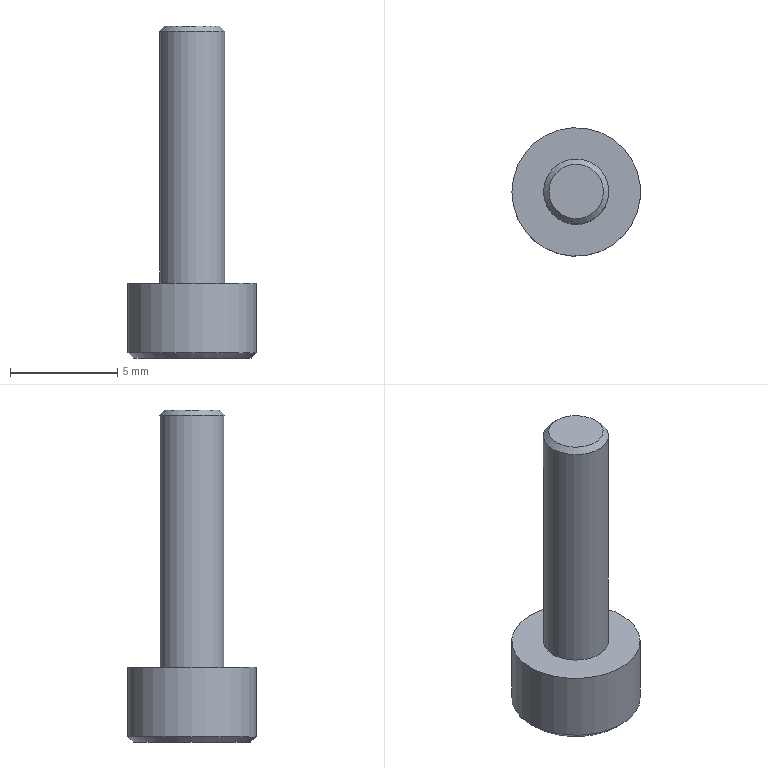Component | NX | SCREW_1 | 1 solid | 14 faces | box 6 x 6 x 15.5 mm | volume 158 mm3 | plane 10 | cylinder 2 | cone 2 | commonest cylinder face diameters 3.045 x1 6 x1
STEP:
#1=CARTESIAN_POINT('',(0.,0.,0.));
#2=DIRECTION('',(0.,0.,1.));
#3=DIRECTION('',(1.,0.,0.));
#4=AXIS2_PLACEMENT_3D('',#1,#2,#3);
#5=CARTESIAN_POINT('',(21.273,19.,-19.));
#6=VERTEX_POINT('',#5);
#7=CARTESIAN_POINT('',(20.,19.,-19.));
#8=DIRECTION('',(0.,0.,1.));
#9=DIRECTION('',(1.,0.,0.));
#10=AXIS2_PLACEMENT_3D('',#7,#8,#9);
#11=CIRCLE('',#10,1.273);
#12=CARTESIAN_POINT('',(20.,19.,-19.));
#13=DIRECTION('',(0.,0.,1.));
#14=DIRECTION('',(1.,0.,0.));
#15=AXIS2_PLACEMENT_3D('',#12,#13,#14);
#16=PLANE('',#15);
#17=CARTESIAN_POINT('',(0.,0.));
#18=DIRECTION('',(1.,0.));
#19=AXIS2_PLACEMENT_2D('',#17,#18);
#20=CIRCLE('',#19,1.273);
#21=(GEOMETRIC_REPRESENTATION_CONTEXT(2)PARAMETRIC_REPRESENTATION_CONTEXT()REPRESENTATION_CONTEXT('',''));
#22=DEFINITIONAL_REPRESENTATION('',(#20),#21);
#23=PCURVE('',#16,#22);
#24=CARTESIAN_POINT('',(20.,19.,-19.25));
#25=DIRECTION('',(0.,0.,-1.));
#26=DIRECTION('',(-1.,0.,0.));
#27=AXIS2_PLACEMENT_3D('',#24,#25,#26);
#28=CONICAL_SURFACE('',#27,1.523,0.7854);
#29=CARTESIAN_POINT('',(9.425,-0.25));
#30=DIRECTION('',(-1.,0.));
#31=VECTOR('',#30,1.);
#32=LINE('',#29,#31);
#33=(GEOMETRIC_REPRESENTATION_CONTEXT(2)PARAMETRIC_REPRESENTATION_CONTEXT()REPRESENTATION_CONTEXT('',''));
#34=DEFINITIONAL_REPRESENTATION('',(#32),#33);
#35=PCURVE('',#28,#34);
#36=SURFACE_CURVE('',#11,(#23,#35),.PCURVE_S1.);
#37=EDGE_CURVE('',#6,#6,#36,.T.);
#38=ORIENTED_EDGE('',*,*,#37,.T.);
#39=EDGE_LOOP('',(#38));
#40=FACE_BOUND('',#39,.T.);
#41=ADVANCED_FACE('',(#40),#16,.T.);
#42=CARTESIAN_POINT('',(21.523,19.,-19.25));
#43=VERTEX_POINT('',#42);
#44=CARTESIAN_POINT('',(18.477,19.,-19.25));
#45=VERTEX_POINT('',#44);
#46=CARTESIAN_POINT('',(20.,19.,-19.25));
#47=DIRECTION('',(0.,0.,-1.));
#48=DIRECTION('',(1.,0.,0.));
#49=AXIS2_PLACEMENT_3D('',#46,#47,#48);
#50=CIRCLE('',#49,1.523);
#51=CARTESIAN_POINT('',(20.,19.,-19.));
#52=DIRECTION('',(0.,0.,-1.));
#53=DIRECTION('',(-1.,0.,0.));
#54=AXIS2_PLACEMENT_3D('',#51,#52,#53);
#55=CYLINDRICAL_SURFACE('',#54,1.523);
#56=CARTESIAN_POINT('',(3.142,0.25));
#57=DIRECTION('',(1.,0.));
#58=VECTOR('',#57,1.);
#59=LINE('',#56,#58);
#60=(GEOMETRIC_REPRESENTATION_CONTEXT(2)PARAMETRIC_REPRESENTATION_CONTEXT()REPRESENTATION_CONTEXT('',''));
#61=DEFINITIONAL_REPRESENTATION('',(#59),#60);
#62=PCURVE('',#55,#61);
#63=CARTESIAN_POINT('',(3.142,-0.));
#64=DIRECTION('',(1.,0.));
#65=VECTOR('',#64,1.);
#66=LINE('',#63,#65);
#67=(GEOMETRIC_REPRESENTATION_CONTEXT(2)PARAMETRIC_REPRESENTATION_CONTEXT()REPRESENTATION_CONTEXT('',''));
#68=DEFINITIONAL_REPRESENTATION('',(#66),#67);
#69=PCURVE('',#28,#68);
#70=SURFACE_CURVE('',#50,(#62,#69),.PCURVE_S1.);
#71=EDGE_CURVE('',#43,#45,#70,.T.);
#72=ORIENTED_EDGE('',*,*,#71,.T.);
#73=CARTESIAN_POINT('',(18.477,19.,-31.));
#74=VERTEX_POINT('',#73);
#75=CARTESIAN_POINT('',(18.477,19.,-19.25));
#76=CARTESIAN_POINT('',(18.477,19.,-31.));
#77=B_SPLINE_CURVE_WITH_KNOTS('',1,(#75,#76),.UNSPECIFIED.,.F.,.F.,(2,2),(0.25,12.),.PIECEWISE_BEZIER_KNOTS.);
#78=CARTESIAN_POINT('',(6.283,0.));
#79=DIRECTION('',(0.,1.));
#80=VECTOR('',#79,1.);
#81=LINE('',#78,#80);
#82=(GEOMETRIC_REPRESENTATION_CONTEXT(2)PARAMETRIC_REPRESENTATION_CONTEXT()REPRESENTATION_CONTEXT('',''));
#83=DEFINITIONAL_REPRESENTATION('',(#81),#82);
#84=PCURVE('',#55,#83);
#85=CARTESIAN_POINT('',(0.,0.));
#86=DIRECTION('',(0.,1.));
#87=VECTOR('',#86,1.);
#88=LINE('',#85,#87);
#89=(GEOMETRIC_REPRESENTATION_CONTEXT(2)PARAMETRIC_REPRESENTATION_CONTEXT()REPRESENTATION_CONTEXT('',''));
#90=DEFINITIONAL_REPRESENTATION('',(#88),#89);
#91=PCURVE('',#55,#90);
#92=SEAM_CURVE('',#77,(#84,#91),.PCURVE_S1.);
#93=EDGE_CURVE('',#45,#74,#92,.T.);
#94=ORIENTED_EDGE('',*,*,#93,.T.);
#95=CARTESIAN_POINT('',(20.,19.,-31.));
#96=DIRECTION('',(0.,0.,1.));
#97=DIRECTION('',(-1.,0.,0.));
#98=AXIS2_PLACEMENT_3D('',#95,#96,#97);
#99=CIRCLE('',#98,1.523);
#100=CARTESIAN_POINT('',(6.283,12.));
#101=DIRECTION('',(-1.,0.));
#102=VECTOR('',#101,1.);
#103=LINE('',#100,#102);
#104=(GEOMETRIC_REPRESENTATION_CONTEXT(2)PARAMETRIC_REPRESENTATION_CONTEXT()REPRESENTATION_CONTEXT('',''));
#105=DEFINITIONAL_REPRESENTATION('',(#103),#104);
#106=PCURVE('',#55,#105);
#107=CARTESIAN_POINT('',(20.,19.,-31.));
#108=DIRECTION('',(0.,0.,1.));
#109=DIRECTION('',(1.,0.,0.));
#110=AXIS2_PLACEMENT_3D('',#107,#108,#109);
#111=PLANE('',#110);
#112=CARTESIAN_POINT('',(0.,0.));
#113=DIRECTION('',(-1.,0.));
#114=AXIS2_PLACEMENT_2D('',#112,#113);
#115=CIRCLE('',#114,1.523);
#116=(GEOMETRIC_REPRESENTATION_CONTEXT(2)PARAMETRIC_REPRESENTATION_CONTEXT()REPRESENTATION_CONTEXT('',''));
#117=DEFINITIONAL_REPRESENTATION('',(#115),#116);
#118=PCURVE('',#111,#117);
#119=SURFACE_CURVE('',#99,(#106,#118),.PCURVE_S1.);
#120=EDGE_CURVE('',#74,#74,#119,.T.);
#121=ORIENTED_EDGE('',*,*,#120,.T.);
#122=ORIENTED_EDGE('',*,*,#93,.F.);
#123=CARTESIAN_POINT('',(20.,19.,-19.25));
#124=DIRECTION('',(0.,0.,-1.));
#125=DIRECTION('',(1.,0.,0.));
#126=AXIS2_PLACEMENT_3D('',#123,#124,#125);
#127=CIRCLE('',#126,1.523);
#128=CARTESIAN_POINT('',(-3.142,0.25));
#129=DIRECTION('',(1.,0.));
#130=VECTOR('',#129,1.);
#131=LINE('',#128,#130);
#132=(GEOMETRIC_REPRESENTATION_CONTEXT(2)PARAMETRIC_REPRESENTATION_CONTEXT()REPRESENTATION_CONTEXT('',''));
#133=DEFINITIONAL_REPRESENTATION('',(#131),#132);
#134=PCURVE('',#55,#133);
#135=CARTESIAN_POINT('',(3.142,-0.));
#136=DIRECTION('',(1.,0.));
#137=VECTOR('',#136,1.);
#138=LINE('',#135,#137);
#139=(GEOMETRIC_REPRESENTATION_CONTEXT(2)PARAMETRIC_REPRESENTATION_CONTEXT()REPRESENTATION_CONTEXT('',''));
#140=DEFINITIONAL_REPRESENTATION('',(#138),#139);
#141=PCURVE('',#28,#140);
#142=SURFACE_CURVE('',#127,(#134,#141),.PCURVE_S1.);
#143=EDGE_CURVE('',#45,#43,#142,.T.);
#144=ORIENTED_EDGE('',*,*,#143,.T.);
#145=EDGE_LOOP('',(#72,#94,#121,#122,#144));
#146=FACE_BOUND('',#145,.T.);
#147=ADVANCED_FACE('',(#146),#55,.T.);
#148=CARTESIAN_POINT('',(17.25,19.,-34.5));
#149=VERTEX_POINT('',#148);
#150=CARTESIAN_POINT('',(20.,19.,-34.5));
#151=DIRECTION('',(0.,0.,-1.));
#152=DIRECTION('',(-1.,0.,0.));
#153=AXIS2_PLACEMENT_3D('',#150,#151,#152);
#154=CIRCLE('',#153,2.75);
#155=CARTESIAN_POINT('',(20.,19.,-34.5));
#156=DIRECTION('',(0.,0.,-1.));
#157=DIRECTION('',(-1.,0.,0.));
#158=AXIS2_PLACEMENT_3D('',#155,#156,#157);
#159=PLANE('',#158);
#160=CARTESIAN_POINT('',(0.,0.));
#161=DIRECTION('',(1.,0.));
#162=AXIS2_PLACEMENT_2D('',#160,#161);
#163=CIRCLE('',#162,2.75);
#164=(GEOMETRIC_REPRESENTATION_CONTEXT(2)PARAMETRIC_REPRESENTATION_CONTEXT()REPRESENTATION_CONTEXT('',''));
#165=DEFINITIONAL_REPRESENTATION('',(#163),#164);
#166=PCURVE('',#159,#165);
#167=CARTESIAN_POINT('',(20.,19.,-34.5));
#168=DIRECTION('',(0.,0.,1.));
#169=DIRECTION('',(1.,0.,0.));
#170=AXIS2_PLACEMENT_3D('',#167,#168,#169);
#171=CONICAL_SURFACE('',#170,2.75,0.7854);
#172=CARTESIAN_POINT('',(9.425,0.));
#173=DIRECTION('',(-1.,0.));
#174=VECTOR('',#173,1.);
#175=LINE('',#172,#174);
#176=(GEOMETRIC_REPRESENTATION_CONTEXT(2)PARAMETRIC_REPRESENTATION_CONTEXT()REPRESENTATION_CONTEXT('',''));
#177=DEFINITIONAL_REPRESENTATION('',(#175),#176);
#178=PCURVE('',#171,#177);
#179=SURFACE_CURVE('',#154,(#166,#178),.PCURVE_S1.);
#180=EDGE_CURVE('',#149,#149,#179,.T.);
#181=ORIENTED_EDGE('',*,*,#180,.T.);
#182=EDGE_LOOP('',(#181));
#183=FACE_BOUND('',#182,.T.);
#184=CARTESIAN_POINT('',(18.845,17.,-34.5));
#185=VERTEX_POINT('',#184);
#186=CARTESIAN_POINT('',(17.691,19.,-34.5));
#187=VERTEX_POINT('',#186);
#188=CARTESIAN_POINT('',(18.845,17.,-34.5));
#189=DIRECTION('',(-0.5,0.866,0.));
#190=VECTOR('',#189,1.);
#191=LINE('',#188,#190);
#192=CARTESIAN_POINT('',(1.155,-2.));
#193=DIRECTION('',(0.5,0.866));
#194=VECTOR('',#193,1.);
#195=LINE('',#192,#194);
#196=(GEOMETRIC_REPRESENTATION_CONTEXT(2)PARAMETRIC_REPRESENTATION_CONTEXT()REPRESENTATION_CONTEXT('',''));
#197=DEFINITIONAL_REPRESENTATION('',(#195),#196);
#198=PCURVE('',#159,#197);
#199=CARTESIAN_POINT('',(18.845,17.,-32.5));
#200=DIRECTION('',(-0.866,-0.5,0.));
#201=DIRECTION('',(-0.5,0.866,0.));
#202=AXIS2_PLACEMENT_3D('',#199,#200,#201);
#203=PLANE('',#202);
#204=CARTESIAN_POINT('',(0.,2.));
#205=DIRECTION('',(1.,0.));
#206=VECTOR('',#205,1.);
#207=LINE('',#204,#206);
#208=(GEOMETRIC_REPRESENTATION_CONTEXT(2)PARAMETRIC_REPRESENTATION_CONTEXT()REPRESENTATION_CONTEXT('',''));
#209=DEFINITIONAL_REPRESENTATION('',(#207),#208);
#210=PCURVE('',#203,#209);
#211=SURFACE_CURVE('',#191,(#198,#210),.PCURVE_S1.);
#212=EDGE_CURVE('',#185,#187,#211,.T.);
#213=ORIENTED_EDGE('',*,*,#212,.F.);
#214=CARTESIAN_POINT('',(21.155,17.,-34.5));
#215=VERTEX_POINT('',#214);
#216=CARTESIAN_POINT('',(21.155,17.,-34.5));
#217=DIRECTION('',(-1.,-0.,0.));
#218=VECTOR('',#217,1.);
#219=LINE('',#216,#218);
#220=CARTESIAN_POINT('',(-1.155,-2.));
#221=DIRECTION('',(1.,-0.));
#222=VECTOR('',#221,1.);
#223=LINE('',#220,#222);
#224=(GEOMETRIC_REPRESENTATION_CONTEXT(2)PARAMETRIC_REPRESENTATION_CONTEXT()REPRESENTATION_CONTEXT('',''));
#225=DEFINITIONAL_REPRESENTATION('',(#223),#224);
#226=PCURVE('',#159,#225);
#227=CARTESIAN_POINT('',(21.155,17.,-32.5));
#228=DIRECTION('',(0.,-1.,0.));
#229=DIRECTION('',(-1.,-0.,0.));
#230=AXIS2_PLACEMENT_3D('',#227,#228,#229);
#231=PLANE('',#230);
#232=CARTESIAN_POINT('',(0.,2.));
#233=DIRECTION('',(1.,0.));
#234=VECTOR('',#233,1.);
#235=LINE('',#232,#234);
#236=(GEOMETRIC_REPRESENTATION_CONTEXT(2)PARAMETRIC_REPRESENTATION_CONTEXT()REPRESENTATION_CONTEXT('',''));
#237=DEFINITIONAL_REPRESENTATION('',(#235),#236);
#238=PCURVE('',#231,#237);
#239=SURFACE_CURVE('',#219,(#226,#238),.PCURVE_S1.);
#240=EDGE_CURVE('',#215,#185,#239,.T.);
#241=ORIENTED_EDGE('',*,*,#240,.F.);
#242=CARTESIAN_POINT('',(22.309,19.,-34.5));
#243=VERTEX_POINT('',#242);
#244=CARTESIAN_POINT('',(22.309,19.,-34.5));
#245=DIRECTION('',(-0.5,-0.866,0.));
#246=VECTOR('',#245,1.);
#247=LINE('',#244,#246);
#248=CARTESIAN_POINT('',(-2.309,0.));
#249=DIRECTION('',(0.5,-0.866));
#250=VECTOR('',#249,1.);
#251=LINE('',#248,#250);
#252=(GEOMETRIC_REPRESENTATION_CONTEXT(2)PARAMETRIC_REPRESENTATION_CONTEXT()REPRESENTATION_CONTEXT('',''));
#253=DEFINITIONAL_REPRESENTATION('',(#251),#252);
#254=PCURVE('',#159,#253);
#255=CARTESIAN_POINT('',(22.309,19.,-32.5));
#256=DIRECTION('',(0.866,-0.5,0.));
#257=DIRECTION('',(-0.5,-0.866,0.));
#258=AXIS2_PLACEMENT_3D('',#255,#256,#257);
#259=PLANE('',#258);
#260=CARTESIAN_POINT('',(0.,2.));
#261=DIRECTION('',(1.,0.));
#262=VECTOR('',#261,1.);
#263=LINE('',#260,#262);
#264=(GEOMETRIC_REPRESENTATION_CONTEXT(2)PARAMETRIC_REPRESENTATION_CONTEXT()REPRESENTATION_CONTEXT('',''));
#265=DEFINITIONAL_REPRESENTATION('',(#263),#264);
#266=PCURVE('',#259,#265);
#267=SURFACE_CURVE('',#247,(#254,#266),.PCURVE_S1.);
#268=EDGE_CURVE('',#243,#215,#267,.T.);
#269=ORIENTED_EDGE('',*,*,#268,.F.);
#270=CARTESIAN_POINT('',(21.155,21.,-34.5));
#271=VERTEX_POINT('',#270);
#272=CARTESIAN_POINT('',(21.155,21.,-34.5));
#273=DIRECTION('',(0.5,-0.866,0.));
#274=VECTOR('',#273,1.);
#275=LINE('',#272,#274);
#276=CARTESIAN_POINT('',(-1.155,2.));
#277=DIRECTION('',(-0.5,-0.866));
#278=VECTOR('',#277,1.);
#279=LINE('',#276,#278);
#280=(GEOMETRIC_REPRESENTATION_CONTEXT(2)PARAMETRIC_REPRESENTATION_CONTEXT()REPRESENTATION_CONTEXT('',''));
#281=DEFINITIONAL_REPRESENTATION('',(#279),#280);
#282=PCURVE('',#159,#281);
#283=CARTESIAN_POINT('',(21.155,21.,-32.5));
#284=DIRECTION('',(0.866,0.5,0.));
#285=DIRECTION('',(0.5,-0.866,0.));
#286=AXIS2_PLACEMENT_3D('',#283,#284,#285);
#287=PLANE('',#286);
#288=CARTESIAN_POINT('',(0.,2.));
#289=DIRECTION('',(1.,0.));
#290=VECTOR('',#289,1.);
#291=LINE('',#288,#290);
#292=(GEOMETRIC_REPRESENTATION_CONTEXT(2)PARAMETRIC_REPRESENTATION_CONTEXT()REPRESENTATION_CONTEXT('',''));
#293=DEFINITIONAL_REPRESENTATION('',(#291),#292);
#294=PCURVE('',#287,#293);
#295=SURFACE_CURVE('',#275,(#282,#294),.PCURVE_S1.);
#296=EDGE_CURVE('',#271,#243,#295,.T.);
#297=ORIENTED_EDGE('',*,*,#296,.F.);
#298=CARTESIAN_POINT('',(18.845,21.,-34.5));
#299=VERTEX_POINT('',#298);
#300=CARTESIAN_POINT('',(18.845,21.,-34.5));
#301=DIRECTION('',(1.,0.,0.));
#302=VECTOR('',#301,1.);
#303=LINE('',#300,#302);
#304=CARTESIAN_POINT('',(1.155,2.));
#305=DIRECTION('',(-1.,0.));
#306=VECTOR('',#305,1.);
#307=LINE('',#304,#306);
#308=(GEOMETRIC_REPRESENTATION_CONTEXT(2)PARAMETRIC_REPRESENTATION_CONTEXT()REPRESENTATION_CONTEXT('',''));
#309=DEFINITIONAL_REPRESENTATION('',(#307),#308);
#310=PCURVE('',#159,#309);
#311=CARTESIAN_POINT('',(18.845,21.,-32.5));
#312=DIRECTION('',(-0.,1.,0.));
#313=DIRECTION('',(1.,0.,0.));
#314=AXIS2_PLACEMENT_3D('',#311,#312,#313);
#315=PLANE('',#314);
#316=CARTESIAN_POINT('',(0.,2.));
#317=DIRECTION('',(1.,0.));
#318=VECTOR('',#317,1.);
#319=LINE('',#316,#318);
#320=(GEOMETRIC_REPRESENTATION_CONTEXT(2)PARAMETRIC_REPRESENTATION_CONTEXT()REPRESENTATION_CONTEXT('',''));
#321=DEFINITIONAL_REPRESENTATION('',(#319),#320);
#322=PCURVE('',#315,#321);
#323=SURFACE_CURVE('',#303,(#310,#322),.PCURVE_S1.);
#324=EDGE_CURVE('',#299,#271,#323,.T.);
#325=ORIENTED_EDGE('',*,*,#324,.F.);
#326=CARTESIAN_POINT('',(17.691,19.,-34.5));
#327=DIRECTION('',(0.5,0.866,0.));
#328=VECTOR('',#327,1.);
#329=LINE('',#326,#328);
#330=CARTESIAN_POINT('',(2.309,0.));
#331=DIRECTION('',(-0.5,0.866));
#332=VECTOR('',#331,1.);
#333=LINE('',#330,#332);
#334=(GEOMETRIC_REPRESENTATION_CONTEXT(2)PARAMETRIC_REPRESENTATION_CONTEXT()REPRESENTATION_CONTEXT('',''));
#335=DEFINITIONAL_REPRESENTATION('',(#333),#334);
#336=PCURVE('',#159,#335);
#337=CARTESIAN_POINT('',(17.691,19.,-32.5));
#338=DIRECTION('',(-0.866,0.5,0.));
#339=DIRECTION('',(0.5,0.866,0.));
#340=AXIS2_PLACEMENT_3D('',#337,#338,#339);
#341=PLANE('',#340);
#342=CARTESIAN_POINT('',(0.,2.));
#343=DIRECTION('',(1.,0.));
#344=VECTOR('',#343,1.);
#345=LINE('',#342,#344);
#346=(GEOMETRIC_REPRESENTATION_CONTEXT(2)PARAMETRIC_REPRESENTATION_CONTEXT()REPRESENTATION_CONTEXT('',''));
#347=DEFINITIONAL_REPRESENTATION('',(#345),#346);
#348=PCURVE('',#341,#347);
#349=SURFACE_CURVE('',#329,(#336,#348),.PCURVE_S1.);
#350=EDGE_CURVE('',#187,#299,#349,.T.);
#351=ORIENTED_EDGE('',*,*,#350,.F.);
#352=EDGE_LOOP('',(#213,#241,#269,#297,#325,#351));
#353=FACE_BOUND('',#352,.T.);
#354=ADVANCED_FACE('',(#183,#353),#159,.T.);
#355=ORIENTED_EDGE('',*,*,#120,.F.);
#356=EDGE_LOOP('',(#355));
#357=FACE_BOUND('',#356,.T.);
#358=CARTESIAN_POINT('',(17.,19.,-31.));
#359=VERTEX_POINT('',#358);
#360=CARTESIAN_POINT('',(20.,19.,-31.));
#361=DIRECTION('',(0.,0.,-1.));
#362=DIRECTION('',(-1.,0.,0.));
#363=AXIS2_PLACEMENT_3D('',#360,#361,#362);
#364=CIRCLE('',#363,3.);
#365=CARTESIAN_POINT('',(-3.,0.));
#366=CARTESIAN_POINT('',(-3.,5.196));
#367=CARTESIAN_POINT('',(1.5,2.598));
#368=CARTESIAN_POINT('',(6.,0.));
#369=CARTESIAN_POINT('',(1.5,-2.598));
#370=CARTESIAN_POINT('',(-3.,-5.196));
#371=CARTESIAN_POINT('',(-3.,0.));
#372=(BOUNDED_CURVE()B_SPLINE_CURVE(2,(#365,#366,#367,#368,#369,#370,#371),.UNSPECIFIED.,.T.,.F.)B_SPLINE_CURVE_WITH_KNOTS((1,2,2,2,2,1),(-2.094,0.,2.094,4.189,6.283,8.378),.UNSPECIFIED.)CURVE()GEOMETRIC_REPRESENTATION_ITEM()RATIONAL_B_SPLINE_CURVE((1.,0.5,1.,0.5,1.,0.5,1.))REPRESENTATION_ITEM(''));
#373=(GEOMETRIC_REPRESENTATION_CONTEXT(2)PARAMETRIC_REPRESENTATION_CONTEXT()REPRESENTATION_CONTEXT('',''));
#374=DEFINITIONAL_REPRESENTATION('',(#372),#373);
#375=PCURVE('',#111,#374);
#376=CARTESIAN_POINT('',(20.,19.,-31.));
#377=DIRECTION('',(0.,0.,-1.));
#378=DIRECTION('',(-1.,0.,0.));
#379=AXIS2_PLACEMENT_3D('',#376,#377,#378);
#380=CYLINDRICAL_SURFACE('',#379,3.);
#381=CARTESIAN_POINT('',(0.,0.));
#382=DIRECTION('',(1.,0.));
#383=VECTOR('',#382,1.);
#384=LINE('',#381,#383);
#385=(GEOMETRIC_REPRESENTATION_CONTEXT(2)PARAMETRIC_REPRESENTATION_CONTEXT()REPRESENTATION_CONTEXT('',''));
#386=DEFINITIONAL_REPRESENTATION('',(#384),#385);
#387=PCURVE('',#380,#386);
#388=SURFACE_CURVE('',#364,(#375,#387),.PCURVE_S1.);
#389=EDGE_CURVE('',#359,#359,#388,.T.);
#390=ORIENTED_EDGE('',*,*,#389,.F.);
#391=EDGE_LOOP('',(#390));
#392=FACE_BOUND('',#391,.T.);
#393=ADVANCED_FACE('',(#357,#392),#111,.T.);
#394=CARTESIAN_POINT('',(17.,19.,-34.25));
#395=VERTEX_POINT('',#394);
#396=CARTESIAN_POINT('',(20.,19.,-34.25));
#397=DIRECTION('',(0.,0.,1.));
#398=DIRECTION('',(-1.,0.,0.));
#399=AXIS2_PLACEMENT_3D('',#396,#397,#398);
#400=CIRCLE('',#399,3.);
#401=CARTESIAN_POINT('',(6.283,3.25));
#402=DIRECTION('',(-1.,0.));
#403=VECTOR('',#402,1.);
#404=LINE('',#401,#403);
#405=(GEOMETRIC_REPRESENTATION_CONTEXT(2)PARAMETRIC_REPRESENTATION_CONTEXT()REPRESENTATION_CONTEXT('',''));
#406=DEFINITIONAL_REPRESENTATION('',(#404),#405);
#407=PCURVE('',#380,#406);
#408=CARTESIAN_POINT('',(3.142,0.25));
#409=DIRECTION('',(1.,0.));
#410=VECTOR('',#409,1.);
#411=LINE('',#408,#410);
#412=(GEOMETRIC_REPRESENTATION_CONTEXT(2)PARAMETRIC_REPRESENTATION_CONTEXT()REPRESENTATION_CONTEXT('',''));
#413=DEFINITIONAL_REPRESENTATION('',(#411),#412);
#414=PCURVE('',#171,#413);
#415=SURFACE_CURVE('',#400,(#407,#414),.PCURVE_S1.);
#416=EDGE_CURVE('',#395,#395,#415,.T.);
#417=ORIENTED_EDGE('',*,*,#416,.T.);
#418=CARTESIAN_POINT('',(17.,19.,-31.));
#419=CARTESIAN_POINT('',(17.,19.,-34.25));
#420=B_SPLINE_CURVE_WITH_KNOTS('',1,(#418,#419),.UNSPECIFIED.,.F.,.F.,(2,2),(0.,3.25),.PIECEWISE_BEZIER_KNOTS.);
#421=CARTESIAN_POINT('',(0.,0.));
#422=DIRECTION('',(0.,1.));
#423=VECTOR('',#422,1.);
#424=LINE('',#421,#423);
#425=(GEOMETRIC_REPRESENTATION_CONTEXT(2)PARAMETRIC_REPRESENTATION_CONTEXT()REPRESENTATION_CONTEXT('',''));
#426=DEFINITIONAL_REPRESENTATION('',(#424),#425);
#427=PCURVE('',#380,#426);
#428=CARTESIAN_POINT('',(6.283,0.));
#429=DIRECTION('',(0.,1.));
#430=VECTOR('',#429,1.);
#431=LINE('',#428,#430);
#432=(GEOMETRIC_REPRESENTATION_CONTEXT(2)PARAMETRIC_REPRESENTATION_CONTEXT()REPRESENTATION_CONTEXT('',''));
#433=DEFINITIONAL_REPRESENTATION('',(#431),#432);
#434=PCURVE('',#380,#433);
#435=SEAM_CURVE('',#420,(#427,#434),.PCURVE_S1.);
#436=EDGE_CURVE('',#359,#395,#435,.T.);
#437=ORIENTED_EDGE('',*,*,#436,.F.);
#438=ORIENTED_EDGE('',*,*,#389,.T.);
#439=ORIENTED_EDGE('',*,*,#436,.T.);
#440=EDGE_LOOP('',(#417,#437,#438,#439));
#441=FACE_BOUND('',#440,.T.);
#442=ADVANCED_FACE('',(#441),#380,.T.);
#443=ORIENTED_EDGE('',*,*,#37,.F.);
#444=CARTESIAN_POINT('',(21.273,19.,-19.));
#445=CARTESIAN_POINT('',(21.523,19.,-19.25));
#446=B_SPLINE_CURVE_WITH_KNOTS('',1,(#444,#445),.UNSPECIFIED.,.F.,.F.,(2,2),(-0.3536,-0.),.PIECEWISE_BEZIER_KNOTS.);
#447=CARTESIAN_POINT('',(9.425,0.));
#448=DIRECTION('',(0.,1.));
#449=VECTOR('',#448,1.);
#450=LINE('',#447,#449);
#451=(GEOMETRIC_REPRESENTATION_CONTEXT(2)PARAMETRIC_REPRESENTATION_CONTEXT()REPRESENTATION_CONTEXT('',''));
#452=DEFINITIONAL_REPRESENTATION('',(#450),#451);
#453=PCURVE('',#28,#452);
#454=CARTESIAN_POINT('',(3.142,0.));
#455=DIRECTION('',(0.,1.));
#456=VECTOR('',#455,1.);
#457=LINE('',#454,#456);
#458=(GEOMETRIC_REPRESENTATION_CONTEXT(2)PARAMETRIC_REPRESENTATION_CONTEXT()REPRESENTATION_CONTEXT('',''));
#459=DEFINITIONAL_REPRESENTATION('',(#457),#458);
#460=PCURVE('',#28,#459);
#461=SEAM_CURVE('',#446,(#453,#460),.PCURVE_S1.);
#462=EDGE_CURVE('',#6,#43,#461,.T.);
#463=ORIENTED_EDGE('',*,*,#462,.T.);
#464=ORIENTED_EDGE('',*,*,#143,.F.);
#465=ORIENTED_EDGE('',*,*,#71,.F.);
#466=ORIENTED_EDGE('',*,*,#462,.F.);
#467=EDGE_LOOP('',(#443,#463,#464,#465,#466));
#468=FACE_BOUND('',#467,.T.);
#469=ADVANCED_FACE('',(#468),#28,.T.);
#470=ORIENTED_EDGE('',*,*,#212,.T.);
#471=CARTESIAN_POINT('',(17.691,19.,-32.5));
#472=VERTEX_POINT('',#471);
#473=CARTESIAN_POINT('',(17.691,19.,-32.5));
#474=DIRECTION('',(0.,0.,1.));
#475=VECTOR('',#474,1.);
#476=LINE('',#473,#475);
#477=CARTESIAN_POINT('',(2.309,0.));
#478=DIRECTION('',(0.,-1.));
#479=VECTOR('',#478,1.);
#480=LINE('',#477,#479);
#481=(GEOMETRIC_REPRESENTATION_CONTEXT(2)PARAMETRIC_REPRESENTATION_CONTEXT()REPRESENTATION_CONTEXT('',''));
#482=DEFINITIONAL_REPRESENTATION('',(#480),#481);
#483=PCURVE('',#203,#482);
#484=CARTESIAN_POINT('',(0.,0.));
#485=DIRECTION('',(0.,-1.));
#486=VECTOR('',#485,1.);
#487=LINE('',#484,#486);
#488=(GEOMETRIC_REPRESENTATION_CONTEXT(2)PARAMETRIC_REPRESENTATION_CONTEXT()REPRESENTATION_CONTEXT('',''));
#489=DEFINITIONAL_REPRESENTATION('',(#487),#488);
#490=PCURVE('',#341,#489);
#491=SURFACE_CURVE('',#476,(#483,#490),.PCURVE_S1.);
#492=EDGE_CURVE('',#187,#472,#491,.T.);
#493=ORIENTED_EDGE('',*,*,#492,.T.);
#494=CARTESIAN_POINT('',(18.845,17.,-32.5));
#495=VERTEX_POINT('',#494);
#496=CARTESIAN_POINT('',(18.845,17.,-32.5));
#497=DIRECTION('',(0.5,-0.866,0.));
#498=VECTOR('',#497,1.);
#499=LINE('',#496,#498);
#500=CARTESIAN_POINT('',(0.,0.));
#501=DIRECTION('',(-1.,0.));
#502=VECTOR('',#501,1.);
#503=LINE('',#500,#502);
#504=(GEOMETRIC_REPRESENTATION_CONTEXT(2)PARAMETRIC_REPRESENTATION_CONTEXT()REPRESENTATION_CONTEXT('',''));
#505=DEFINITIONAL_REPRESENTATION('',(#503),#504);
#506=PCURVE('',#203,#505);
#507=CARTESIAN_POINT('',(20.,19.,-32.5));
#508=DIRECTION('',(0.,0.,-1.));
#509=DIRECTION('',(-1.,0.,0.));
#510=AXIS2_PLACEMENT_3D('',#507,#508,#509);
#511=PLANE('',#510);
#512=CARTESIAN_POINT('',(1.155,-2.));
#513=DIRECTION('',(-0.5,-0.866));
#514=VECTOR('',#513,1.);
#515=LINE('',#512,#514);
#516=(GEOMETRIC_REPRESENTATION_CONTEXT(2)PARAMETRIC_REPRESENTATION_CONTEXT()REPRESENTATION_CONTEXT('',''));
#517=DEFINITIONAL_REPRESENTATION('',(#515),#516);
#518=PCURVE('',#511,#517);
#519=SURFACE_CURVE('',#499,(#506,#518),.PCURVE_S1.);
#520=EDGE_CURVE('',#472,#495,#519,.T.);
#521=ORIENTED_EDGE('',*,*,#520,.T.);
#522=CARTESIAN_POINT('',(18.845,17.,-32.5));
#523=DIRECTION('',(0.,0.,1.));
#524=VECTOR('',#523,1.);
#525=LINE('',#522,#524);
#526=CARTESIAN_POINT('',(0.,0.));
#527=DIRECTION('',(0.,-1.));
#528=VECTOR('',#527,1.);
#529=LINE('',#526,#528);
#530=(GEOMETRIC_REPRESENTATION_CONTEXT(2)PARAMETRIC_REPRESENTATION_CONTEXT()REPRESENTATION_CONTEXT('',''));
#531=DEFINITIONAL_REPRESENTATION('',(#529),#530);
#532=PCURVE('',#203,#531);
#533=CARTESIAN_POINT('',(2.309,0.));
#534=DIRECTION('',(0.,-1.));
#535=VECTOR('',#534,1.);
#536=LINE('',#533,#535);
#537=(GEOMETRIC_REPRESENTATION_CONTEXT(2)PARAMETRIC_REPRESENTATION_CONTEXT()REPRESENTATION_CONTEXT('',''));
#538=DEFINITIONAL_REPRESENTATION('',(#536),#537);
#539=PCURVE('',#231,#538);
#540=SURFACE_CURVE('',#525,(#532,#539),.PCURVE_S1.);
#541=EDGE_CURVE('',#185,#495,#540,.T.);
#542=ORIENTED_EDGE('',*,*,#541,.F.);
#543=EDGE_LOOP('',(#470,#493,#521,#542));
#544=FACE_BOUND('',#543,.T.);
#545=ADVANCED_FACE('',(#544),#203,.F.);
#546=ORIENTED_EDGE('',*,*,#350,.T.);
#547=CARTESIAN_POINT('',(18.845,21.,-32.5));
#548=VERTEX_POINT('',#547);
#549=CARTESIAN_POINT('',(18.845,21.,-32.5));
#550=DIRECTION('',(0.,0.,1.));
#551=VECTOR('',#550,1.);
#552=LINE('',#549,#551);
#553=CARTESIAN_POINT('',(2.309,0.));
#554=DIRECTION('',(0.,-1.));
#555=VECTOR('',#554,1.);
#556=LINE('',#553,#555);
#557=(GEOMETRIC_REPRESENTATION_CONTEXT(2)PARAMETRIC_REPRESENTATION_CONTEXT()REPRESENTATION_CONTEXT('',''));
#558=DEFINITIONAL_REPRESENTATION('',(#556),#557);
#559=PCURVE('',#341,#558);
#560=CARTESIAN_POINT('',(0.,0.));
#561=DIRECTION('',(0.,-1.));
#562=VECTOR('',#561,1.);
#563=LINE('',#560,#562);
#564=(GEOMETRIC_REPRESENTATION_CONTEXT(2)PARAMETRIC_REPRESENTATION_CONTEXT()REPRESENTATION_CONTEXT('',''));
#565=DEFINITIONAL_REPRESENTATION('',(#563),#564);
#566=PCURVE('',#315,#565);
#567=SURFACE_CURVE('',#552,(#559,#566),.PCURVE_S1.);
#568=EDGE_CURVE('',#299,#548,#567,.T.);
#569=ORIENTED_EDGE('',*,*,#568,.T.);
#570=CARTESIAN_POINT('',(17.691,19.,-32.5));
#571=DIRECTION('',(-0.5,-0.866,0.));
#572=VECTOR('',#571,1.);
#573=LINE('',#570,#572);
#574=CARTESIAN_POINT('',(0.,0.));
#575=DIRECTION('',(-1.,0.));
#576=VECTOR('',#575,1.);
#577=LINE('',#574,#576);
#578=(GEOMETRIC_REPRESENTATION_CONTEXT(2)PARAMETRIC_REPRESENTATION_CONTEXT()REPRESENTATION_CONTEXT('',''));
#579=DEFINITIONAL_REPRESENTATION('',(#577),#578);
#580=PCURVE('',#341,#579);
#581=CARTESIAN_POINT('',(2.309,0.));
#582=DIRECTION('',(0.5,-0.866));
#583=VECTOR('',#582,1.);
#584=LINE('',#581,#583);
#585=(GEOMETRIC_REPRESENTATION_CONTEXT(2)PARAMETRIC_REPRESENTATION_CONTEXT()REPRESENTATION_CONTEXT('',''));
#586=DEFINITIONAL_REPRESENTATION('',(#584),#585);
#587=PCURVE('',#511,#586);
#588=SURFACE_CURVE('',#573,(#580,#587),.PCURVE_S1.);
#589=EDGE_CURVE('',#548,#472,#588,.T.);
#590=ORIENTED_EDGE('',*,*,#589,.T.);
#591=ORIENTED_EDGE('',*,*,#492,.F.);
#592=EDGE_LOOP('',(#546,#569,#590,#591));
#593=FACE_BOUND('',#592,.T.);
#594=ADVANCED_FACE('',(#593),#341,.F.);
#595=ORIENTED_EDGE('',*,*,#324,.T.);
#596=CARTESIAN_POINT('',(21.155,21.,-32.5));
#597=VERTEX_POINT('',#596);
#598=CARTESIAN_POINT('',(21.155,21.,-32.5));
#599=DIRECTION('',(0.,0.,1.));
#600=VECTOR('',#599,1.);
#601=LINE('',#598,#600);
#602=CARTESIAN_POINT('',(2.309,0.));
#603=DIRECTION('',(0.,-1.));
#604=VECTOR('',#603,1.);
#605=LINE('',#602,#604);
#606=(GEOMETRIC_REPRESENTATION_CONTEXT(2)PARAMETRIC_REPRESENTATION_CONTEXT()REPRESENTATION_CONTEXT('',''));
#607=DEFINITIONAL_REPRESENTATION('',(#605),#606);
#608=PCURVE('',#315,#607);
#609=CARTESIAN_POINT('',(0.,0.));
#610=DIRECTION('',(0.,-1.));
#611=VECTOR('',#610,1.);
#612=LINE('',#609,#611);
#613=(GEOMETRIC_REPRESENTATION_CONTEXT(2)PARAMETRIC_REPRESENTATION_CONTEXT()REPRESENTATION_CONTEXT('',''));
#614=DEFINITIONAL_REPRESENTATION('',(#612),#613);
#615=PCURVE('',#287,#614);
#616=SURFACE_CURVE('',#601,(#608,#615),.PCURVE_S1.);
#617=EDGE_CURVE('',#271,#597,#616,.T.);
#618=ORIENTED_EDGE('',*,*,#617,.T.);
#619=CARTESIAN_POINT('',(18.845,21.,-32.5));
#620=DIRECTION('',(-1.,-0.,0.));
#621=VECTOR('',#620,1.);
#622=LINE('',#619,#621);
#623=CARTESIAN_POINT('',(0.,0.));
#624=DIRECTION('',(-1.,0.));
#625=VECTOR('',#624,1.);
#626=LINE('',#623,#625);
#627=(GEOMETRIC_REPRESENTATION_CONTEXT(2)PARAMETRIC_REPRESENTATION_CONTEXT()REPRESENTATION_CONTEXT('',''));
#628=DEFINITIONAL_REPRESENTATION('',(#626),#627);
#629=PCURVE('',#315,#628);
#630=CARTESIAN_POINT('',(1.155,2.));
#631=DIRECTION('',(1.,-0.));
#632=VECTOR('',#631,1.);
#633=LINE('',#630,#632);
#634=(GEOMETRIC_REPRESENTATION_CONTEXT(2)PARAMETRIC_REPRESENTATION_CONTEXT()REPRESENTATION_CONTEXT('',''));
#635=DEFINITIONAL_REPRESENTATION('',(#633),#634);
#636=PCURVE('',#511,#635);
#637=SURFACE_CURVE('',#622,(#629,#636),.PCURVE_S1.);
#638=EDGE_CURVE('',#597,#548,#637,.T.);
#639=ORIENTED_EDGE('',*,*,#638,.T.);
#640=ORIENTED_EDGE('',*,*,#568,.F.);
#641=EDGE_LOOP('',(#595,#618,#639,#640));
#642=FACE_BOUND('',#641,.T.);
#643=ADVANCED_FACE('',(#642),#315,.F.);
#644=ORIENTED_EDGE('',*,*,#296,.T.);
#645=CARTESIAN_POINT('',(22.309,19.,-32.5));
#646=VERTEX_POINT('',#645);
#647=CARTESIAN_POINT('',(22.309,19.,-32.5));
#648=DIRECTION('',(0.,0.,1.));
#649=VECTOR('',#648,1.);
#650=LINE('',#647,#649);
#651=CARTESIAN_POINT('',(2.309,0.));
#652=DIRECTION('',(0.,-1.));
#653=VECTOR('',#652,1.);
#654=LINE('',#651,#653);
#655=(GEOMETRIC_REPRESENTATION_CONTEXT(2)PARAMETRIC_REPRESENTATION_CONTEXT()REPRESENTATION_CONTEXT('',''));
#656=DEFINITIONAL_REPRESENTATION('',(#654),#655);
#657=PCURVE('',#287,#656);
#658=CARTESIAN_POINT('',(0.,0.));
#659=DIRECTION('',(0.,-1.));
#660=VECTOR('',#659,1.);
#661=LINE('',#658,#660);
#662=(GEOMETRIC_REPRESENTATION_CONTEXT(2)PARAMETRIC_REPRESENTATION_CONTEXT()REPRESENTATION_CONTEXT('',''));
#663=DEFINITIONAL_REPRESENTATION('',(#661),#662);
#664=PCURVE('',#259,#663);
#665=SURFACE_CURVE('',#650,(#657,#664),.PCURVE_S1.);
#666=EDGE_CURVE('',#243,#646,#665,.T.);
#667=ORIENTED_EDGE('',*,*,#666,.T.);
#668=CARTESIAN_POINT('',(21.155,21.,-32.5));
#669=DIRECTION('',(-0.5,0.866,0.));
#670=VECTOR('',#669,1.);
#671=LINE('',#668,#670);
#672=CARTESIAN_POINT('',(0.,0.));
#673=DIRECTION('',(-1.,0.));
#674=VECTOR('',#673,1.);
#675=LINE('',#672,#674);
#676=(GEOMETRIC_REPRESENTATION_CONTEXT(2)PARAMETRIC_REPRESENTATION_CONTEXT()REPRESENTATION_CONTEXT('',''));
#677=DEFINITIONAL_REPRESENTATION('',(#675),#676);
#678=PCURVE('',#287,#677);
#679=CARTESIAN_POINT('',(-1.155,2.));
#680=DIRECTION('',(0.5,0.866));
#681=VECTOR('',#680,1.);
#682=LINE('',#679,#681);
#683=(GEOMETRIC_REPRESENTATION_CONTEXT(2)PARAMETRIC_REPRESENTATION_CONTEXT()REPRESENTATION_CONTEXT('',''));
#684=DEFINITIONAL_REPRESENTATION('',(#682),#683);
#685=PCURVE('',#511,#684);
#686=SURFACE_CURVE('',#671,(#678,#685),.PCURVE_S1.);
#687=EDGE_CURVE('',#646,#597,#686,.T.);
#688=ORIENTED_EDGE('',*,*,#687,.T.);
#689=ORIENTED_EDGE('',*,*,#617,.F.);
#690=EDGE_LOOP('',(#644,#667,#688,#689));
#691=FACE_BOUND('',#690,.T.);
#692=ADVANCED_FACE('',(#691),#287,.F.);
#693=ORIENTED_EDGE('',*,*,#268,.T.);
#694=CARTESIAN_POINT('',(21.155,17.,-32.5));
#695=VERTEX_POINT('',#694);
#696=CARTESIAN_POINT('',(21.155,17.,-32.5));
#697=DIRECTION('',(0.,0.,1.));
#698=VECTOR('',#697,1.);
#699=LINE('',#696,#698);
#700=CARTESIAN_POINT('',(2.309,0.));
#701=DIRECTION('',(0.,-1.));
#702=VECTOR('',#701,1.);
#703=LINE('',#700,#702);
#704=(GEOMETRIC_REPRESENTATION_CONTEXT(2)PARAMETRIC_REPRESENTATION_CONTEXT()REPRESENTATION_CONTEXT('',''));
#705=DEFINITIONAL_REPRESENTATION('',(#703),#704);
#706=PCURVE('',#259,#705);
#707=CARTESIAN_POINT('',(0.,0.));
#708=DIRECTION('',(0.,-1.));
#709=VECTOR('',#708,1.);
#710=LINE('',#707,#709);
#711=(GEOMETRIC_REPRESENTATION_CONTEXT(2)PARAMETRIC_REPRESENTATION_CONTEXT()REPRESENTATION_CONTEXT('',''));
#712=DEFINITIONAL_REPRESENTATION('',(#710),#711);
#713=PCURVE('',#231,#712);
#714=SURFACE_CURVE('',#699,(#706,#713),.PCURVE_S1.);
#715=EDGE_CURVE('',#215,#695,#714,.T.);
#716=ORIENTED_EDGE('',*,*,#715,.T.);
#717=CARTESIAN_POINT('',(22.309,19.,-32.5));
#718=DIRECTION('',(0.5,0.866,0.));
#719=VECTOR('',#718,1.);
#720=LINE('',#717,#719);
#721=CARTESIAN_POINT('',(0.,0.));
#722=DIRECTION('',(-1.,0.));
#723=VECTOR('',#722,1.);
#724=LINE('',#721,#723);
#725=(GEOMETRIC_REPRESENTATION_CONTEXT(2)PARAMETRIC_REPRESENTATION_CONTEXT()REPRESENTATION_CONTEXT('',''));
#726=DEFINITIONAL_REPRESENTATION('',(#724),#725);
#727=PCURVE('',#259,#726);
#728=CARTESIAN_POINT('',(-2.309,0.));
#729=DIRECTION('',(-0.5,0.866));
#730=VECTOR('',#729,1.);
#731=LINE('',#728,#730);
#732=(GEOMETRIC_REPRESENTATION_CONTEXT(2)PARAMETRIC_REPRESENTATION_CONTEXT()REPRESENTATION_CONTEXT('',''));
#733=DEFINITIONAL_REPRESENTATION('',(#731),#732);
#734=PCURVE('',#511,#733);
#735=SURFACE_CURVE('',#720,(#727,#734),.PCURVE_S1.);
#736=EDGE_CURVE('',#695,#646,#735,.T.);
#737=ORIENTED_EDGE('',*,*,#736,.T.);
#738=ORIENTED_EDGE('',*,*,#666,.F.);
#739=EDGE_LOOP('',(#693,#716,#737,#738));
#740=FACE_BOUND('',#739,.T.);
#741=ADVANCED_FACE('',(#740),#259,.F.);
#742=ORIENTED_EDGE('',*,*,#240,.T.);
#743=ORIENTED_EDGE('',*,*,#541,.T.);
#744=CARTESIAN_POINT('',(21.155,17.,-32.5));
#745=DIRECTION('',(1.,0.,0.));
#746=VECTOR('',#745,1.);
#747=LINE('',#744,#746);
#748=CARTESIAN_POINT('',(0.,0.));
#749=DIRECTION('',(-1.,0.));
#750=VECTOR('',#749,1.);
#751=LINE('',#748,#750);
#752=(GEOMETRIC_REPRESENTATION_CONTEXT(2)PARAMETRIC_REPRESENTATION_CONTEXT()REPRESENTATION_CONTEXT('',''));
#753=DEFINITIONAL_REPRESENTATION('',(#751),#752);
#754=PCURVE('',#231,#753);
#755=CARTESIAN_POINT('',(-1.155,-2.));
#756=DIRECTION('',(-1.,0.));
#757=VECTOR('',#756,1.);
#758=LINE('',#755,#757);
#759=(GEOMETRIC_REPRESENTATION_CONTEXT(2)PARAMETRIC_REPRESENTATION_CONTEXT()REPRESENTATION_CONTEXT('',''));
#760=DEFINITIONAL_REPRESENTATION('',(#758),#759);
#761=PCURVE('',#511,#760);
#762=SURFACE_CURVE('',#747,(#754,#761),.PCURVE_S1.);
#763=EDGE_CURVE('',#495,#695,#762,.T.);
#764=ORIENTED_EDGE('',*,*,#763,.T.);
#765=ORIENTED_EDGE('',*,*,#715,.F.);
#766=EDGE_LOOP('',(#742,#743,#764,#765));
#767=FACE_BOUND('',#766,.T.);
#768=ADVANCED_FACE('',(#767),#231,.F.);
#769=ORIENTED_EDGE('',*,*,#520,.F.);
#770=ORIENTED_EDGE('',*,*,#589,.F.);
#771=ORIENTED_EDGE('',*,*,#638,.F.);
#772=ORIENTED_EDGE('',*,*,#687,.F.);
#773=ORIENTED_EDGE('',*,*,#736,.F.);
#774=ORIENTED_EDGE('',*,*,#763,.F.);
#775=EDGE_LOOP('',(#769,#770,#771,#772,#773,#774));
#776=FACE_BOUND('',#775,.T.);
#777=ADVANCED_FACE('',(#776),#511,.T.);
#778=ORIENTED_EDGE('',*,*,#416,.F.);
#779=CARTESIAN_POINT('',(17.25,19.,-34.5));
#780=CARTESIAN_POINT('',(17.,19.,-34.25));
#781=B_SPLINE_CURVE_WITH_KNOTS('',1,(#779,#780),.UNSPECIFIED.,.F.,.F.,(2,2),(0.,0.3536),.PIECEWISE_BEZIER_KNOTS.);
#782=CARTESIAN_POINT('',(3.142,0.));
#783=DIRECTION('',(0.,1.));
#784=VECTOR('',#783,1.);
#785=LINE('',#782,#784);
#786=(GEOMETRIC_REPRESENTATION_CONTEXT(2)PARAMETRIC_REPRESENTATION_CONTEXT()REPRESENTATION_CONTEXT('',''));
#787=DEFINITIONAL_REPRESENTATION('',(#785),#786);
#788=PCURVE('',#171,#787);
#789=CARTESIAN_POINT('',(9.425,0.));
#790=DIRECTION('',(0.,1.));
#791=VECTOR('',#790,1.);
#792=LINE('',#789,#791);
#793=(GEOMETRIC_REPRESENTATION_CONTEXT(2)PARAMETRIC_REPRESENTATION_CONTEXT()REPRESENTATION_CONTEXT('',''));
#794=DEFINITIONAL_REPRESENTATION('',(#792),#793);
#795=PCURVE('',#171,#794);
#796=SEAM_CURVE('',#781,(#788,#795),.PCURVE_S1.);
#797=EDGE_CURVE('',#149,#395,#796,.T.);
#798=ORIENTED_EDGE('',*,*,#797,.F.);
#799=ORIENTED_EDGE('',*,*,#180,.F.);
#800=ORIENTED_EDGE('',*,*,#797,.T.);
#801=EDGE_LOOP('',(#778,#798,#799,#800));
#802=FACE_BOUND('',#801,.T.);
#803=ADVANCED_FACE('',(#802),#171,.T.);
#804=CLOSED_SHELL('',(#41,#147,#354,#393,#442,#469,#545,#594,#643,#692,#741,#768,#777,#803));
#805=MANIFOLD_SOLID_BREP('',#804);
#806=(LENGTH_UNIT()NAMED_UNIT(*)SI_UNIT(.MILLI.,.METRE.));
#807=UNCERTAINTY_MEASURE_WITH_UNIT(LENGTH_MEASURE(0.000002),#806,'','');
#808=(NAMED_UNIT(*)PLANE_ANGLE_UNIT()SI_UNIT($,.RADIAN.));
#809=(NAMED_UNIT(*)SI_UNIT($,.STERADIAN.)SOLID_ANGLE_UNIT());
#810=(GEOMETRIC_REPRESENTATION_CONTEXT(3)GLOBAL_UNCERTAINTY_ASSIGNED_CONTEXT((#807))GLOBAL_UNIT_ASSIGNED_CONTEXT((#806,#808,#809))REPRESENTATION_CONTEXT('',''));
#811=ADVANCED_BREP_SHAPE_REPRESENTATION('',(#4,#805),#810);